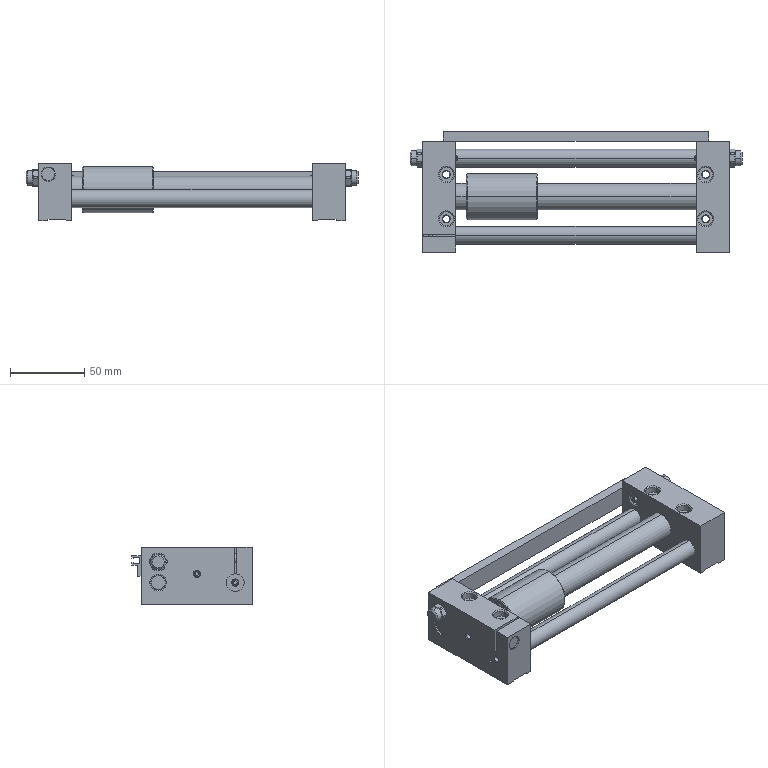Component | SolidWorks | BearingLiftingModule-1_RMT16X100S_0_+_CS1-G-2-1_RMT-16X100-S(0)-G-2_rod-1 | 1 solid | 246 faces | volume 234105 mm3 | plane 90 | cylinder 86 | cone 66 | torus 4 | commonest cylinder face diameters 12 x18 4.917 x10 5.5 x8 9.5 x8 10 x8 10.5 x4 6.5 x4 18 x4